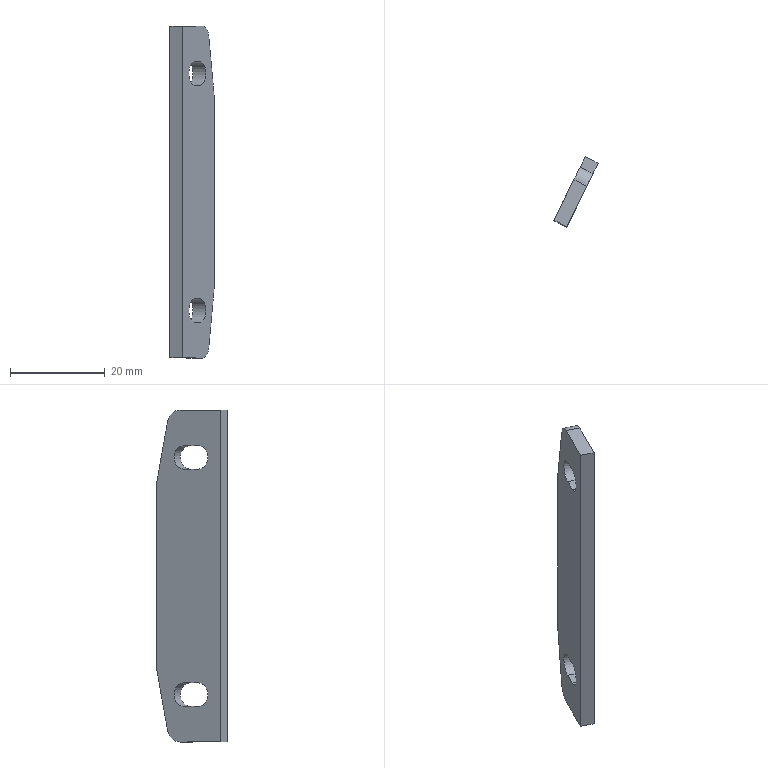Component | SolidWorks | YX-04-109GluePaperFeedingExpansionPlate-1 | 1 solid | 18 faces | box 9.35 x 14.77 x 70 mm | volume 2800 mm3 | plane 12 | cylinder 6 | commonest cylinder face diameters 5 x4 6 x2 | material Delrin
build123d program:
from build123d import *

# Parameters (mm, degrees)
BOSS_EXTRUDE1_DEPTH = 3


with BuildPart() as part:
    # Sketch1 → Boss-Extrude1 (new body)
    with BuildSketch(Plane.XY.offset(1.5)):
        with BuildLine():
            Line((35, -7.5), (35, 2.041))
            ThreePointArc((35, 2.041), (34.32, 3.943), (32.588, 4.982))
            Line((32.588, 4.982), (20, 7.5))
            Line((20, 7.5), (-20, 7.5))
            Line((-20, 7.5), (-32.588, 4.982))
            ThreePointArc((-32.588, 4.982), (-34.32, 3.943), (-35, 2.041))
            Line((-35, 2.041), (-35, -7.5))
            Line((-35, -7.5), (35, -7.5))
        make_face()
        with BuildLine():
            Line((-27.5, -2), (-27.5, 1))
            ThreePointArc((-27.5, 1), (-25, 3.5), (-22.5, 1))
            Line((-22.5, 1), (-22.5, -2))
            ThreePointArc((-22.5, -2), (-25, -4.5), (-27.5, -2))
        make_face(mode=Mode.SUBTRACT)
        with BuildLine():
            Line((22.5, -2), (22.5, 1))
            ThreePointArc((22.5, 1), (25, 3.5), (27.5, 1))
            Line((27.5, 1), (27.5, -2))
            ThreePointArc((27.5, -2), (25, -4.5), (22.5, -2))
        make_face(mode=Mode.SUBTRACT)
    extrude(amount=-BOSS_EXTRUDE1_DEPTH)


solid = part.part

# Placed as in the assembly
solid = solid.moved(Location((-89.137, 35.001, 147), (90, 63.609, -90)))
STEP:
#1=CARTESIAN_POINT('',(-3.693,1.14,4.409));
#2=VERTEX_POINT('',#1);
#3=CARTESIAN_POINT('',(-3.693,1.14,7.165));
#4=VERTEX_POINT('',#3);
#5=CARTESIAN_POINT('',(-3.693,1.14,4.409));
#6=DIRECTION('',(0.,0.,1.));
#7=VECTOR('',#6,39.37);
#8=LINE('',#5,#7);
#9=EDGE_CURVE('',#2,#4,#8,.T.);
#10=ORIENTED_EDGE('',*,*,#9,.F.);
#11=CARTESIAN_POINT('',(-3.588,1.087,4.409));
#12=VERTEX_POINT('',#11);
#13=CARTESIAN_POINT('',(-3.588,1.087,4.409));
#14=DIRECTION('',(-0.8958,0.4445,-0.));
#15=VECTOR('',#14,39.37);
#16=LINE('',#13,#15);
#17=EDGE_CURVE('',#12,#2,#16,.T.);
#18=ORIENTED_EDGE('',*,*,#17,.F.);
#19=CARTESIAN_POINT('',(-3.588,1.087,7.165));
#20=VERTEX_POINT('',#19);
#21=CARTESIAN_POINT('',(-3.588,1.087,4.409));
#22=DIRECTION('',(0.,0.,1.));
#23=VECTOR('',#22,39.37);
#24=LINE('',#21,#23);
#25=EDGE_CURVE('',#12,#20,#24,.T.);
#26=ORIENTED_EDGE('',*,*,#25,.T.);
#27=CARTESIAN_POINT('',(-3.588,1.087,7.165));
#28=DIRECTION('',(-0.8958,0.4445,-0.));
#29=VECTOR('',#28,39.37);
#30=LINE('',#27,#29);
#31=EDGE_CURVE('',#20,#4,#30,.T.);
#32=ORIENTED_EDGE('',*,*,#31,.T.);
#33=EDGE_LOOP('',(#10,#18,#26,#32));
#34=FACE_OUTER_BOUND('',#33,.T.);
#35=CARTESIAN_POINT('',(-3.588,1.087,4.409));
#36=DIRECTION('',(-0.4445,-0.8958,0.));
#37=DIRECTION('',(0.8958,-0.4445,0.));
#38=AXIS2_PLACEMENT_3D('',#35,#36,#37);
#39=PLANE('',#38);
#40=ADVANCED_FACE('',(#34),#39,.T.);
#41=CARTESIAN_POINT('',(-3.527,1.476,4.409));
#42=VERTEX_POINT('',#41);
#43=CARTESIAN_POINT('',(-3.527,1.476,4.409));
#44=DIRECTION('',(-0.4445,-0.8958,0.));
#45=VECTOR('',#44,39.37);
#46=LINE('',#43,#45);
#47=EDGE_CURVE('',#42,#2,#46,.T.);
#48=ORIENTED_EDGE('',*,*,#47,.F.);
#49=CARTESIAN_POINT('',(-3.421,1.424,4.409));
#50=VERTEX_POINT('',#49);
#51=CARTESIAN_POINT('',(-3.421,1.424,4.409));
#52=DIRECTION('',(-0.8958,0.4445,-0.));
#53=VECTOR('',#52,39.37);
#54=LINE('',#51,#53);
#55=EDGE_CURVE('',#50,#42,#54,.T.);
#56=ORIENTED_EDGE('',*,*,#55,.F.);
#57=CARTESIAN_POINT('',(-3.421,1.424,4.409));
#58=DIRECTION('',(-0.4445,-0.8958,0.));
#59=VECTOR('',#58,39.37);
#60=LINE('',#57,#59);
#61=EDGE_CURVE('',#50,#12,#60,.T.);
#62=ORIENTED_EDGE('',*,*,#61,.T.);
#63=ORIENTED_EDGE('',*,*,#17,.T.);
#64=EDGE_LOOP('',(#48,#56,#62,#63));
#65=FACE_OUTER_BOUND('',#64,.T.);
#66=CARTESIAN_POINT('',(-3.421,1.424,4.409));
#67=DIRECTION('',(-0.,-0.,-1.));
#68=DIRECTION('',(-0.8958,0.4445,-0.));
#69=AXIS2_PLACEMENT_3D('',#66,#67,#68);
#70=PLANE('',#69);
#71=ADVANCED_FACE('',(#65),#70,.T.);
#72=CARTESIAN_POINT('',(-3.475,1.58,4.504));
#73=VERTEX_POINT('',#72);
#74=CARTESIAN_POINT('',(-3.527,1.476,4.528));
#75=DIRECTION('',(-0.8958,0.4445,-0.));
#76=DIRECTION('',(0.,0.,1.));
#77=AXIS2_PLACEMENT_3D('',#74,#75,#76);
#78=CIRCLE('',#77,0.1181);
#79=EDGE_CURVE('',#73,#42,#78,.T.);
#80=ORIENTED_EDGE('',*,*,#79,.F.);
#81=CARTESIAN_POINT('',(-3.369,1.527,4.504));
#82=VERTEX_POINT('',#81);
#83=CARTESIAN_POINT('',(-3.369,1.527,4.504));
#84=DIRECTION('',(-0.8958,0.4445,-0.));
#85=VECTOR('',#84,39.37);
#86=LINE('',#83,#85);
#87=EDGE_CURVE('',#82,#73,#86,.T.);
#88=ORIENTED_EDGE('',*,*,#87,.F.);
#89=CARTESIAN_POINT('',(-3.421,1.424,4.528));
#90=DIRECTION('',(-0.8958,0.4445,-0.));
#91=DIRECTION('',(0.,0.,1.));
#92=AXIS2_PLACEMENT_3D('',#89,#90,#91);
#93=CIRCLE('',#92,0.1181);
#94=EDGE_CURVE('',#82,#50,#93,.T.);
#95=ORIENTED_EDGE('',*,*,#94,.T.);
#96=ORIENTED_EDGE('',*,*,#55,.T.);
#97=EDGE_LOOP('',(#80,#88,#95,#96));
#98=FACE_OUTER_BOUND('',#97,.T.);
#99=CARTESIAN_POINT('',(-3.421,1.424,4.528));
#100=DIRECTION('',(-0.8958,0.4445,-0.));
#101=DIRECTION('',(0.,0.,1.));
#102=AXIS2_PLACEMENT_3D('',#99,#100,#101);
#103=CYLINDRICAL_SURFACE('',#102,0.1181);
#104=ADVANCED_FACE('',(#98),#103,.T.);
#105=CARTESIAN_POINT('',(-3.431,1.669,5.));
#106=VERTEX_POINT('',#105);
#107=CARTESIAN_POINT('',(-3.431,1.669,5.));
#108=DIRECTION('',(-0.08717,-0.1757,-0.9806));
#109=VECTOR('',#108,39.37);
#110=LINE('',#107,#109);
#111=EDGE_CURVE('',#106,#73,#110,.T.);
#112=ORIENTED_EDGE('',*,*,#111,.F.);
#113=CARTESIAN_POINT('',(-3.325,1.616,5.));
#114=VERTEX_POINT('',#113);
#115=CARTESIAN_POINT('',(-3.325,1.616,5.));
#116=DIRECTION('',(-0.8958,0.4445,-0.));
#117=VECTOR('',#116,39.37);
#118=LINE('',#115,#117);
#119=EDGE_CURVE('',#114,#106,#118,.T.);
#120=ORIENTED_EDGE('',*,*,#119,.F.);
#121=CARTESIAN_POINT('',(-3.325,1.616,5.));
#122=DIRECTION('',(-0.08717,-0.1757,-0.9806));
#123=VECTOR('',#122,39.37);
#124=LINE('',#121,#123);
#125=EDGE_CURVE('',#114,#82,#124,.T.);
#126=ORIENTED_EDGE('',*,*,#125,.T.);
#127=ORIENTED_EDGE('',*,*,#87,.T.);
#128=EDGE_LOOP('',(#112,#120,#126,#127));
#129=FACE_OUTER_BOUND('',#128,.T.);
#130=CARTESIAN_POINT('',(-3.325,1.616,5.));
#131=DIRECTION('',(0.4359,0.8784,-0.1961));
#132=DIRECTION('',(-0.08717,-0.1757,-0.9806));
#133=AXIS2_PLACEMENT_3D('',#130,#131,#132);
#134=PLANE('',#133);
#135=ADVANCED_FACE('',(#129),#134,.T.);
#136=CARTESIAN_POINT('',(-3.431,1.669,6.575));
#137=VERTEX_POINT('',#136);
#138=CARTESIAN_POINT('',(-3.431,1.669,6.575));
#139=DIRECTION('',(-0.,-0.,-1.));
#140=VECTOR('',#139,39.37);
#141=LINE('',#138,#140);
#142=EDGE_CURVE('',#137,#106,#141,.T.);
#143=ORIENTED_EDGE('',*,*,#142,.F.);
#144=CARTESIAN_POINT('',(-3.325,1.616,6.575));
#145=VERTEX_POINT('',#144);
#146=CARTESIAN_POINT('',(-3.325,1.616,6.575));
#147=DIRECTION('',(-0.8958,0.4445,-0.));
#148=VECTOR('',#147,39.37);
#149=LINE('',#146,#148);
#150=EDGE_CURVE('',#145,#137,#149,.T.);
#151=ORIENTED_EDGE('',*,*,#150,.F.);
#152=CARTESIAN_POINT('',(-3.325,1.616,6.575));
#153=DIRECTION('',(-0.,-0.,-1.));
#154=VECTOR('',#153,39.37);
#155=LINE('',#152,#154);
#156=EDGE_CURVE('',#145,#114,#155,.T.);
#157=ORIENTED_EDGE('',*,*,#156,.T.);
#158=ORIENTED_EDGE('',*,*,#119,.T.);
#159=EDGE_LOOP('',(#143,#151,#157,#158));
#160=FACE_OUTER_BOUND('',#159,.T.);
#161=CARTESIAN_POINT('',(-3.325,1.616,6.575));
#162=DIRECTION('',(0.4445,0.8958,-0.));
#163=DIRECTION('',(-0.,-0.,-1.));
#164=AXIS2_PLACEMENT_3D('',#161,#162,#163);
#165=PLANE('',#164);
#166=ADVANCED_FACE('',(#160),#165,.T.);
#167=CARTESIAN_POINT('',(-3.475,1.58,7.07));
#168=VERTEX_POINT('',#167);
#169=CARTESIAN_POINT('',(-3.475,1.58,7.07));
#170=DIRECTION('',(0.08717,0.1757,-0.9806));
#171=VECTOR('',#170,39.37);
#172=LINE('',#169,#171);
#173=EDGE_CURVE('',#168,#137,#172,.T.);
#174=ORIENTED_EDGE('',*,*,#173,.F.);
#175=CARTESIAN_POINT('',(-3.369,1.527,7.07));
#176=VERTEX_POINT('',#175);
#177=CARTESIAN_POINT('',(-3.369,1.527,7.07));
#178=DIRECTION('',(-0.8958,0.4445,-0.));
#179=VECTOR('',#178,39.37);
#180=LINE('',#177,#179);
#181=EDGE_CURVE('',#176,#168,#180,.T.);
#182=ORIENTED_EDGE('',*,*,#181,.F.);
#183=CARTESIAN_POINT('',(-3.369,1.527,7.07));
#184=DIRECTION('',(0.08717,0.1757,-0.9806));
#185=VECTOR('',#184,39.37);
#186=LINE('',#183,#185);
#187=EDGE_CURVE('',#176,#145,#186,.T.);
#188=ORIENTED_EDGE('',*,*,#187,.T.);
#189=ORIENTED_EDGE('',*,*,#150,.T.);
#190=EDGE_LOOP('',(#174,#182,#188,#189));
#191=FACE_OUTER_BOUND('',#190,.T.);
#192=CARTESIAN_POINT('',(-3.369,1.527,7.07));
#193=DIRECTION('',(0.4359,0.8784,0.1961));
#194=DIRECTION('',(0.08717,0.1757,-0.9806));
#195=AXIS2_PLACEMENT_3D('',#192,#193,#194);
#196=PLANE('',#195);
#197=ADVANCED_FACE('',(#191),#196,.T.);
#198=CARTESIAN_POINT('',(-3.527,1.476,7.165));
#199=VERTEX_POINT('',#198);
#200=CARTESIAN_POINT('',(-3.527,1.476,7.047));
#201=DIRECTION('',(-0.8958,0.4445,-0.));
#202=DIRECTION('',(0.,0.,1.));
#203=AXIS2_PLACEMENT_3D('',#200,#201,#202);
#204=CIRCLE('',#203,0.1181);
#205=EDGE_CURVE('',#199,#168,#204,.T.);
#206=ORIENTED_EDGE('',*,*,#205,.F.);
#207=CARTESIAN_POINT('',(-3.421,1.424,7.165));
#208=VERTEX_POINT('',#207);
#209=CARTESIAN_POINT('',(-3.421,1.424,7.165));
#210=DIRECTION('',(-0.8958,0.4445,-0.));
#211=VECTOR('',#210,39.37);
#212=LINE('',#209,#211);
#213=EDGE_CURVE('',#208,#199,#212,.T.);
#214=ORIENTED_EDGE('',*,*,#213,.F.);
#215=CARTESIAN_POINT('',(-3.421,1.424,7.047));
#216=DIRECTION('',(-0.8958,0.4445,-0.));
#217=DIRECTION('',(0.,0.,1.));
#218=AXIS2_PLACEMENT_3D('',#215,#216,#217);
#219=CIRCLE('',#218,0.1181);
#220=EDGE_CURVE('',#208,#176,#219,.T.);
#221=ORIENTED_EDGE('',*,*,#220,.T.);
#222=ORIENTED_EDGE('',*,*,#181,.T.);
#223=EDGE_LOOP('',(#206,#214,#221,#222));
#224=FACE_OUTER_BOUND('',#223,.T.);
#225=CARTESIAN_POINT('',(-3.421,1.424,7.047));
#226=DIRECTION('',(-0.8958,0.4445,-0.));
#227=DIRECTION('',(0.,0.,1.));
#228=AXIS2_PLACEMENT_3D('',#225,#226,#227);
#229=CYLINDRICAL_SURFACE('',#228,0.1181);
#230=ADVANCED_FACE('',(#224),#229,.T.);
#231=CARTESIAN_POINT('',(-3.693,1.14,7.165));
#232=DIRECTION('',(0.4445,0.8958,-0.));
#233=VECTOR('',#232,39.37);
#234=LINE('',#231,#233);
#235=EDGE_CURVE('',#4,#199,#234,.T.);
#236=ORIENTED_EDGE('',*,*,#235,.F.);
#237=ORIENTED_EDGE('',*,*,#31,.F.);
#238=CARTESIAN_POINT('',(-3.588,1.087,7.165));
#239=DIRECTION('',(0.4445,0.8958,-0.));
#240=VECTOR('',#239,39.37);
#241=LINE('',#238,#240);
#242=EDGE_CURVE('',#20,#208,#241,.T.);
#243=ORIENTED_EDGE('',*,*,#242,.T.);
#244=ORIENTED_EDGE('',*,*,#213,.T.);
#245=EDGE_LOOP('',(#236,#237,#243,#244));
#246=FACE_OUTER_BOUND('',#245,.T.);
#247=CARTESIAN_POINT('',(-3.588,1.087,7.165));
#248=DIRECTION('',(0.,0.,1.));
#249=DIRECTION('',(0.8958,-0.4445,0.));
#250=AXIS2_PLACEMENT_3D('',#247,#248,#249);
#251=PLANE('',#250);
#252=ADVANCED_FACE('',(#246),#251,.T.);
#253=CARTESIAN_POINT('',(-3.439,1.387,6.673));
#254=VERTEX_POINT('',#253);
#255=CARTESIAN_POINT('',(-3.491,1.281,6.673));
#256=VERTEX_POINT('',#255);
#257=CARTESIAN_POINT('',(-3.491,1.281,6.673));
#258=DIRECTION('',(-0.4445,-0.8958,0.));
#259=VECTOR('',#258,39.37);
#260=LINE('',#257,#259);
#261=EDGE_CURVE('',#254,#256,#260,.T.);
#262=ORIENTED_EDGE('',*,*,#261,.T.);
#263=CARTESIAN_POINT('',(-3.491,1.281,6.87));
#264=VERTEX_POINT('',#263);
#265=CARTESIAN_POINT('',(-3.491,1.281,6.772));
#266=DIRECTION('',(-0.8958,0.4445,-0.));
#267=DIRECTION('',(0.,0.,-1.));
#268=AXIS2_PLACEMENT_3D('',#265,#266,#267);
#269=CIRCLE('',#268,0.09843);
#270=EDGE_CURVE('',#256,#264,#269,.T.);
#271=ORIENTED_EDGE('',*,*,#270,.T.);
#272=CARTESIAN_POINT('',(-3.439,1.387,6.87));
#273=VERTEX_POINT('',#272);
#274=CARTESIAN_POINT('',(-3.439,1.387,6.87));
#275=DIRECTION('',(0.4445,0.8958,-0.));
#276=VECTOR('',#275,39.37);
#277=LINE('',#274,#276);
#278=EDGE_CURVE('',#264,#273,#277,.T.);
#279=ORIENTED_EDGE('',*,*,#278,.T.);
#280=CARTESIAN_POINT('',(-3.439,1.387,6.772));
#281=DIRECTION('',(-0.8958,0.4445,-0.));
#282=DIRECTION('',(0.,0.,-1.));
#283=AXIS2_PLACEMENT_3D('',#280,#281,#282);
#284=CIRCLE('',#283,0.09843);
#285=EDGE_CURVE('',#273,#254,#284,.T.);
#286=ORIENTED_EDGE('',*,*,#285,.T.);
#287=EDGE_LOOP('',(#262,#271,#279,#286));
#288=FACE_BOUND('',#287,.T.);
#289=CARTESIAN_POINT('',(-3.439,1.387,4.705));
#290=VERTEX_POINT('',#289);
#291=CARTESIAN_POINT('',(-3.491,1.281,4.705));
#292=VERTEX_POINT('',#291);
#293=CARTESIAN_POINT('',(-3.491,1.281,4.705));
#294=DIRECTION('',(-0.4445,-0.8958,0.));
#295=VECTOR('',#294,39.37);
#296=LINE('',#293,#295);
#297=EDGE_CURVE('',#290,#292,#296,.T.);
#298=ORIENTED_EDGE('',*,*,#297,.T.);
#299=CARTESIAN_POINT('',(-3.491,1.281,4.902));
#300=VERTEX_POINT('',#299);
#301=CARTESIAN_POINT('',(-3.491,1.281,4.803));
#302=DIRECTION('',(-0.8958,0.4445,-0.));
#303=DIRECTION('',(0.,0.,-1.));
#304=AXIS2_PLACEMENT_3D('',#301,#302,#303);
#305=CIRCLE('',#304,0.09843);
#306=EDGE_CURVE('',#292,#300,#305,.T.);
#307=ORIENTED_EDGE('',*,*,#306,.T.);
#308=CARTESIAN_POINT('',(-3.439,1.387,4.902));
#309=VERTEX_POINT('',#308);
#310=CARTESIAN_POINT('',(-3.439,1.387,4.902));
#311=DIRECTION('',(0.4445,0.8958,-0.));
#312=VECTOR('',#311,39.37);
#313=LINE('',#310,#312);
#314=EDGE_CURVE('',#300,#309,#313,.T.);
#315=ORIENTED_EDGE('',*,*,#314,.T.);
#316=CARTESIAN_POINT('',(-3.439,1.387,4.803));
#317=DIRECTION('',(-0.8958,0.4445,-0.));
#318=DIRECTION('',(0.,0.,-1.));
#319=AXIS2_PLACEMENT_3D('',#316,#317,#318);
#320=CIRCLE('',#319,0.09843);
#321=EDGE_CURVE('',#309,#290,#320,.T.);
#322=ORIENTED_EDGE('',*,*,#321,.T.);
#323=EDGE_LOOP('',(#298,#307,#315,#322));
#324=FACE_BOUND('',#323,.T.);
#325=ORIENTED_EDGE('',*,*,#25,.F.);
#326=ORIENTED_EDGE('',*,*,#61,.F.);
#327=ORIENTED_EDGE('',*,*,#94,.F.);
#328=ORIENTED_EDGE('',*,*,#125,.F.);
#329=ORIENTED_EDGE('',*,*,#156,.F.);
#330=ORIENTED_EDGE('',*,*,#187,.F.);
#331=ORIENTED_EDGE('',*,*,#220,.F.);
#332=ORIENTED_EDGE('',*,*,#242,.F.);
#333=EDGE_LOOP('',(#325,#326,#327,#328,#329,#330,#331,#332));
#334=FACE_OUTER_BOUND('',#333,.T.);
#335=CARTESIAN_POINT('',(-3.421,1.424,7.047));
#336=DIRECTION('',(-0.8958,0.4445,-0.));
#337=DIRECTION('',(0.,0.,1.));
#338=AXIS2_PLACEMENT_3D('',#335,#336,#337);
#339=PLANE('',#338);
#340=ADVANCED_FACE('',(#288,#324,#334),#339,.F.);
#341=CARTESIAN_POINT('',(-3.597,1.334,6.673));
#342=VERTEX_POINT('',#341);
#343=CARTESIAN_POINT('',(-3.597,1.334,6.87));
#344=VERTEX_POINT('',#343);
#345=CARTESIAN_POINT('',(-3.597,1.334,6.772));
#346=DIRECTION('',(-0.8958,0.4445,-0.));
#347=DIRECTION('',(0.,0.,-1.));
#348=AXIS2_PLACEMENT_3D('',#345,#346,#347);
#349=CIRCLE('',#348,0.09843);
#350=EDGE_CURVE('',#342,#344,#349,.T.);
#351=ORIENTED_EDGE('',*,*,#350,.F.);
#352=CARTESIAN_POINT('',(-3.545,1.44,6.673));
#353=VERTEX_POINT('',#352);
#354=CARTESIAN_POINT('',(-3.597,1.334,6.673));
#355=DIRECTION('',(-0.4445,-0.8958,0.));
#356=VECTOR('',#355,39.37);
#357=LINE('',#354,#356);
#358=EDGE_CURVE('',#353,#342,#357,.T.);
#359=ORIENTED_EDGE('',*,*,#358,.F.);
#360=CARTESIAN_POINT('',(-3.545,1.44,6.87));
#361=VERTEX_POINT('',#360);
#362=CARTESIAN_POINT('',(-3.545,1.44,6.772));
#363=DIRECTION('',(-0.8958,0.4445,-0.));
#364=DIRECTION('',(0.,0.,-1.));
#365=AXIS2_PLACEMENT_3D('',#362,#363,#364);
#366=CIRCLE('',#365,0.09843);
#367=EDGE_CURVE('',#361,#353,#366,.T.);
#368=ORIENTED_EDGE('',*,*,#367,.F.);
#369=CARTESIAN_POINT('',(-3.545,1.44,6.87));
#370=DIRECTION('',(0.4445,0.8958,-0.));
#371=VECTOR('',#370,39.37);
#372=LINE('',#369,#371);
#373=EDGE_CURVE('',#344,#361,#372,.T.);
#374=ORIENTED_EDGE('',*,*,#373,.F.);
#375=EDGE_LOOP('',(#351,#359,#368,#374));
#376=FACE_BOUND('',#375,.T.);
#377=CARTESIAN_POINT('',(-3.597,1.334,4.705));
#378=VERTEX_POINT('',#377);
#379=CARTESIAN_POINT('',(-3.597,1.334,4.902));
#380=VERTEX_POINT('',#379);
#381=CARTESIAN_POINT('',(-3.597,1.334,4.803));
#382=DIRECTION('',(-0.8958,0.4445,-0.));
#383=DIRECTION('',(0.,0.,-1.));
#384=AXIS2_PLACEMENT_3D('',#381,#382,#383);
#385=CIRCLE('',#384,0.09843);
#386=EDGE_CURVE('',#378,#380,#385,.T.);
#387=ORIENTED_EDGE('',*,*,#386,.F.);
#388=CARTESIAN_POINT('',(-3.545,1.44,4.705));
#389=VERTEX_POINT('',#388);
#390=CARTESIAN_POINT('',(-3.597,1.334,4.705));
#391=DIRECTION('',(-0.4445,-0.8958,0.));
#392=VECTOR('',#391,39.37);
#393=LINE('',#390,#392);
#394=EDGE_CURVE('',#389,#378,#393,.T.);
#395=ORIENTED_EDGE('',*,*,#394,.F.);
#396=CARTESIAN_POINT('',(-3.545,1.44,4.902));
#397=VERTEX_POINT('',#396);
#398=CARTESIAN_POINT('',(-3.545,1.44,4.803));
#399=DIRECTION('',(-0.8958,0.4445,-0.));
#400=DIRECTION('',(0.,0.,-1.));
#401=AXIS2_PLACEMENT_3D('',#398,#399,#400);
#402=CIRCLE('',#401,0.09843);
#403=EDGE_CURVE('',#397,#389,#402,.T.);
#404=ORIENTED_EDGE('',*,*,#403,.F.);
#405=CARTESIAN_POINT('',(-3.545,1.44,4.902));
#406=DIRECTION('',(0.4445,0.8958,-0.));
#407=VECTOR('',#406,39.37);
#408=LINE('',#405,#407);
#409=EDGE_CURVE('',#380,#397,#408,.T.);
#410=ORIENTED_EDGE('',*,*,#409,.F.);
#411=EDGE_LOOP('',(#387,#395,#404,#410));
#412=FACE_BOUND('',#411,.T.);
#413=ORIENTED_EDGE('',*,*,#9,.T.);
#414=ORIENTED_EDGE('',*,*,#235,.T.);
#415=ORIENTED_EDGE('',*,*,#205,.T.);
#416=ORIENTED_EDGE('',*,*,#173,.T.);
#417=ORIENTED_EDGE('',*,*,#142,.T.);
#418=ORIENTED_EDGE('',*,*,#111,.T.);
#419=ORIENTED_EDGE('',*,*,#79,.T.);
#420=ORIENTED_EDGE('',*,*,#47,.T.);
#421=EDGE_LOOP('',(#413,#414,#415,#416,#417,#418,#419,#420));
#422=FACE_OUTER_BOUND('',#421,.T.);
#423=CARTESIAN_POINT('',(-3.527,1.476,7.047));
#424=DIRECTION('',(-0.8958,0.4445,-0.));
#425=DIRECTION('',(0.,0.,1.));
#426=AXIS2_PLACEMENT_3D('',#423,#424,#425);
#427=PLANE('',#426);
#428=ADVANCED_FACE('',(#376,#412,#422),#427,.T.);
#429=ORIENTED_EDGE('',*,*,#386,.T.);
#430=CARTESIAN_POINT('',(-3.491,1.281,4.902));
#431=DIRECTION('',(-0.8958,0.4445,-0.));
#432=VECTOR('',#431,39.37);
#433=LINE('',#430,#432);
#434=EDGE_CURVE('',#300,#380,#433,.T.);
#435=ORIENTED_EDGE('',*,*,#434,.F.);
#436=ORIENTED_EDGE('',*,*,#306,.F.);
#437=CARTESIAN_POINT('',(-3.491,1.281,4.705));
#438=DIRECTION('',(-0.8958,0.4445,-0.));
#439=VECTOR('',#438,39.37);
#440=LINE('',#437,#439);
#441=EDGE_CURVE('',#292,#378,#440,.T.);
#442=ORIENTED_EDGE('',*,*,#441,.T.);
#443=EDGE_LOOP('',(#429,#435,#436,#442));
#444=FACE_OUTER_BOUND('',#443,.T.);
#445=CARTESIAN_POINT('',(-3.491,1.281,4.803));
#446=DIRECTION('',(-0.8958,0.4445,-0.));
#447=DIRECTION('',(0.,0.,1.));
#448=AXIS2_PLACEMENT_3D('',#445,#446,#447);
#449=CYLINDRICAL_SURFACE('',#448,0.09843);
#450=ADVANCED_FACE('',(#444),#449,.F.);
#451=ORIENTED_EDGE('',*,*,#394,.T.);
#452=ORIENTED_EDGE('',*,*,#441,.F.);
#453=ORIENTED_EDGE('',*,*,#297,.F.);
#454=CARTESIAN_POINT('',(-3.439,1.387,4.705));
#455=DIRECTION('',(-0.8958,0.4445,-0.));
#456=VECTOR('',#455,39.37);
#457=LINE('',#454,#456);
#458=EDGE_CURVE('',#290,#389,#457,.T.);
#459=ORIENTED_EDGE('',*,*,#458,.T.);
#460=EDGE_LOOP('',(#451,#452,#453,#459));
#461=FACE_OUTER_BOUND('',#460,.T.);
#462=CARTESIAN_POINT('',(-3.491,1.281,4.705));
#463=DIRECTION('',(-0.,-0.,-1.));
#464=DIRECTION('',(-0.8958,0.4445,-0.));
#465=AXIS2_PLACEMENT_3D('',#462,#463,#464);
#466=PLANE('',#465);
#467=ADVANCED_FACE('',(#461),#466,.F.);
#468=ORIENTED_EDGE('',*,*,#403,.T.);
#469=ORIENTED_EDGE('',*,*,#458,.F.);
#470=ORIENTED_EDGE('',*,*,#321,.F.);
#471=CARTESIAN_POINT('',(-3.439,1.387,4.902));
#472=DIRECTION('',(-0.8958,0.4445,-0.));
#473=VECTOR('',#472,39.37);
#474=LINE('',#471,#473);
#475=EDGE_CURVE('',#309,#397,#474,.T.);
#476=ORIENTED_EDGE('',*,*,#475,.T.);
#477=EDGE_LOOP('',(#468,#469,#470,#476));
#478=FACE_OUTER_BOUND('',#477,.T.);
#479=CARTESIAN_POINT('',(-3.439,1.387,4.803));
#480=DIRECTION('',(-0.8958,0.4445,-0.));
#481=DIRECTION('',(0.,0.,1.));
#482=AXIS2_PLACEMENT_3D('',#479,#480,#481);
#483=CYLINDRICAL_SURFACE('',#482,0.09843);
#484=ADVANCED_FACE('',(#478),#483,.F.);
#485=ORIENTED_EDGE('',*,*,#409,.T.);
#486=ORIENTED_EDGE('',*,*,#475,.F.);
#487=ORIENTED_EDGE('',*,*,#314,.F.);
#488=ORIENTED_EDGE('',*,*,#434,.T.);
#489=EDGE_LOOP('',(#485,#486,#487,#488));
#490=FACE_OUTER_BOUND('',#489,.T.);
#491=CARTESIAN_POINT('',(-3.439,1.387,4.902));
#492=DIRECTION('',(0.,0.,1.));
#493=DIRECTION('',(0.8958,-0.4445,0.));
#494=AXIS2_PLACEMENT_3D('',#491,#492,#493);
#495=PLANE('',#494);
#496=ADVANCED_FACE('',(#490),#495,.F.);
#497=ORIENTED_EDGE('',*,*,#350,.T.);
#498=CARTESIAN_POINT('',(-3.491,1.281,6.87));
#499=DIRECTION('',(-0.8958,0.4445,-0.));
#500=VECTOR('',#499,39.37);
#501=LINE('',#498,#500);
#502=EDGE_CURVE('',#264,#344,#501,.T.);
#503=ORIENTED_EDGE('',*,*,#502,.F.);
#504=ORIENTED_EDGE('',*,*,#270,.F.);
#505=CARTESIAN_POINT('',(-3.491,1.281,6.673));
#506=DIRECTION('',(-0.8958,0.4445,-0.));
#507=VECTOR('',#506,39.37);
#508=LINE('',#505,#507);
#509=EDGE_CURVE('',#256,#342,#508,.T.);
#510=ORIENTED_EDGE('',*,*,#509,.T.);
#511=EDGE_LOOP('',(#497,#503,#504,#510));
#512=FACE_OUTER_BOUND('',#511,.T.);
#513=CARTESIAN_POINT('',(-3.491,1.281,6.772));
#514=DIRECTION('',(-0.8958,0.4445,-0.));
#515=DIRECTION('',(0.,0.,1.));
#516=AXIS2_PLACEMENT_3D('',#513,#514,#515);
#517=CYLINDRICAL_SURFACE('',#516,0.09843);
#518=ADVANCED_FACE('',(#512),#517,.F.);
#519=ORIENTED_EDGE('',*,*,#358,.T.);
#520=ORIENTED_EDGE('',*,*,#509,.F.);
#521=ORIENTED_EDGE('',*,*,#261,.F.);
#522=CARTESIAN_POINT('',(-3.439,1.387,6.673));
#523=DIRECTION('',(-0.8958,0.4445,-0.));
#524=VECTOR('',#523,39.37);
#525=LINE('',#522,#524);
#526=EDGE_CURVE('',#254,#353,#525,.T.);
#527=ORIENTED_EDGE('',*,*,#526,.T.);
#528=EDGE_LOOP('',(#519,#520,#521,#527));
#529=FACE_OUTER_BOUND('',#528,.T.);
#530=CARTESIAN_POINT('',(-3.491,1.281,6.673));
#531=DIRECTION('',(-0.,-0.,-1.));
#532=DIRECTION('',(-0.8958,0.4445,-0.));
#533=AXIS2_PLACEMENT_3D('',#530,#531,#532);
#534=PLANE('',#533);
#535=ADVANCED_FACE('',(#529),#534,.F.);
#536=ORIENTED_EDGE('',*,*,#367,.T.);
#537=ORIENTED_EDGE('',*,*,#526,.F.);
#538=ORIENTED_EDGE('',*,*,#285,.F.);
#539=CARTESIAN_POINT('',(-3.439,1.387,6.87));
#540=DIRECTION('',(-0.8958,0.4445,-0.));
#541=VECTOR('',#540,39.37);
#542=LINE('',#539,#541);
#543=EDGE_CURVE('',#273,#361,#542,.T.);
#544=ORIENTED_EDGE('',*,*,#543,.T.);
#545=EDGE_LOOP('',(#536,#537,#538,#544));
#546=FACE_OUTER_BOUND('',#545,.T.);
#547=CARTESIAN_POINT('',(-3.439,1.387,6.772));
#548=DIRECTION('',(-0.8958,0.4445,-0.));
#549=DIRECTION('',(0.,0.,1.));
#550=AXIS2_PLACEMENT_3D('',#547,#548,#549);
#551=CYLINDRICAL_SURFACE('',#550,0.09843);
#552=ADVANCED_FACE('',(#546),#551,.F.);
#553=ORIENTED_EDGE('',*,*,#373,.T.);
#554=ORIENTED_EDGE('',*,*,#543,.F.);
#555=ORIENTED_EDGE('',*,*,#278,.F.);
#556=ORIENTED_EDGE('',*,*,#502,.T.);
#557=EDGE_LOOP('',(#553,#554,#555,#556));
#558=FACE_OUTER_BOUND('',#557,.T.);
#559=CARTESIAN_POINT('',(-3.439,1.387,6.87));
#560=DIRECTION('',(0.,0.,1.));
#561=DIRECTION('',(0.8958,-0.4445,0.));
#562=AXIS2_PLACEMENT_3D('',#559,#560,#561);
#563=PLANE('',#562);
#564=ADVANCED_FACE('',(#558),#563,.F.);
#565=CLOSED_SHELL('',(#40,#71,#104,#135,#166,#197,#230,#252,#340,#428,#450,#467,#484,#496,#518,#535,#552,#564));
#566=MANIFOLD_SOLID_BREP('',#565);
#567=CARTESIAN_POINT('',(0.,0.,0.));
#568=DIRECTION('',(0.,0.,1.));
#569=DIRECTION('',(1.,0.,0.));
#570=AXIS2_PLACEMENT_3D('',#567,#568,#569);
#571=(LENGTH_UNIT()NAMED_UNIT(*)SI_UNIT($,.METRE.));
#572=LENGTH_MEASURE_WITH_UNIT(LENGTH_MEASURE(0.0254),#571);
#573=DIMENSIONAL_EXPONENTS(1.,0.,0.,0.,0.,0.,0.);
#574=(CONVERSION_BASED_UNIT('',#572)LENGTH_UNIT()NAMED_UNIT(#573));
#575=UNCERTAINTY_MEASURE_WITH_UNIT(LENGTH_MEASURE(0.00001),#574,'','');
#576=(NAMED_UNIT(*)PLANE_ANGLE_UNIT()SI_UNIT($,.RADIAN.));
#577=(NAMED_UNIT(*)SI_UNIT($,.STERADIAN.)SOLID_ANGLE_UNIT());
#578=(GEOMETRIC_REPRESENTATION_CONTEXT(3)GLOBAL_UNCERTAINTY_ASSIGNED_CONTEXT((#575))GLOBAL_UNIT_ASSIGNED_CONTEXT((#574,#576,#577))REPRESENTATION_CONTEXT('',''));
#579=ADVANCED_BREP_SHAPE_REPRESENTATION('',(#566,#570),#578);
#580=COLOUR_RGB('',0.7922,0.8196,0.9333);
#581=FILL_AREA_STYLE_COLOUR('',#580);
#582=FILL_AREA_STYLE('',(#581));
#583=SURFACE_STYLE_FILL_AREA(#582);
#584=SURFACE_SIDE_STYLE('',(#583));
#585=SURFACE_STYLE_USAGE(.BOTH.,#584);
#586=PRESENTATION_STYLE_ASSIGNMENT((#585));
#587=STYLED_ITEM('',(#586),#566);
#588=PRESENTATION_LAYER_ASSIGNMENT('','',(#587));
#589=(LENGTH_UNIT()NAMED_UNIT(*)SI_UNIT($,.METRE.));
#590=LENGTH_MEASURE_WITH_UNIT(LENGTH_MEASURE(0.0254),#589);
#591=DIMENSIONAL_EXPONENTS(1.,0.,0.,0.,0.,0.,0.);
#592=(CONVERSION_BASED_UNIT('',#590)LENGTH_UNIT()NAMED_UNIT(#591));
#593=UNCERTAINTY_MEASURE_WITH_UNIT(LENGTH_MEASURE(0.00001),#592,'','');
#594=(NAMED_UNIT(*)PLANE_ANGLE_UNIT()SI_UNIT($,.RADIAN.));
#595=(NAMED_UNIT(*)SI_UNIT($,.STERADIAN.)SOLID_ANGLE_UNIT());
#596=(GEOMETRIC_REPRESENTATION_CONTEXT(3)GLOBAL_UNCERTAINTY_ASSIGNED_CONTEXT((#593))GLOBAL_UNIT_ASSIGNED_CONTEXT((#592,#594,#595))REPRESENTATION_CONTEXT('',''));
#597=MECHANICAL_DESIGN_GEOMETRIC_PRESENTATION_REPRESENTATION('',(#587),#596);